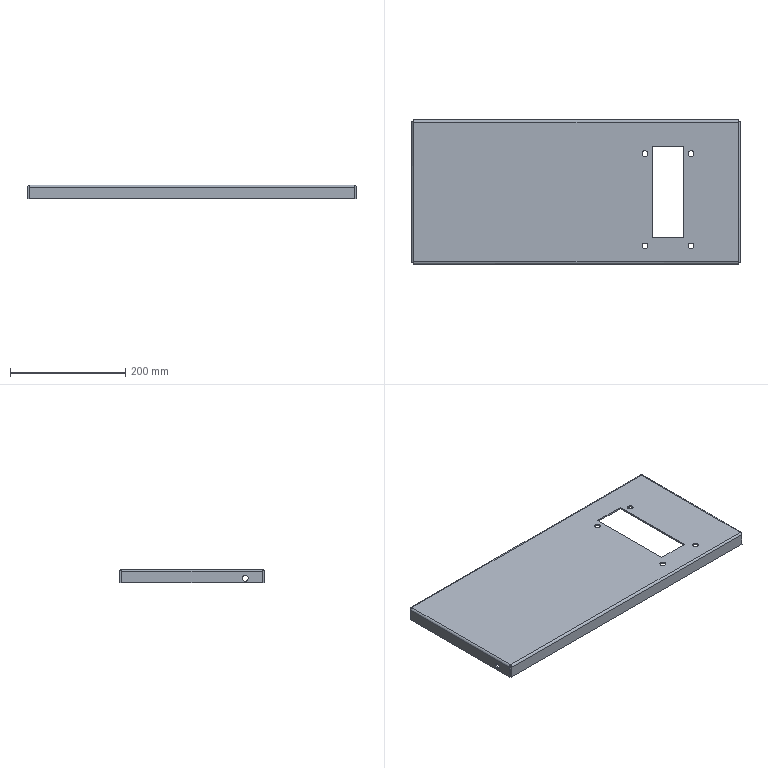Component | SolidWorks | ActuatorGasket-1 | 1 solid | 54 faces | volume 456659 mm3 | plane 26 | cylinder 20 | spline 8 | commonest cylinder face diameters 10 x12 2 x4 7.5 x4